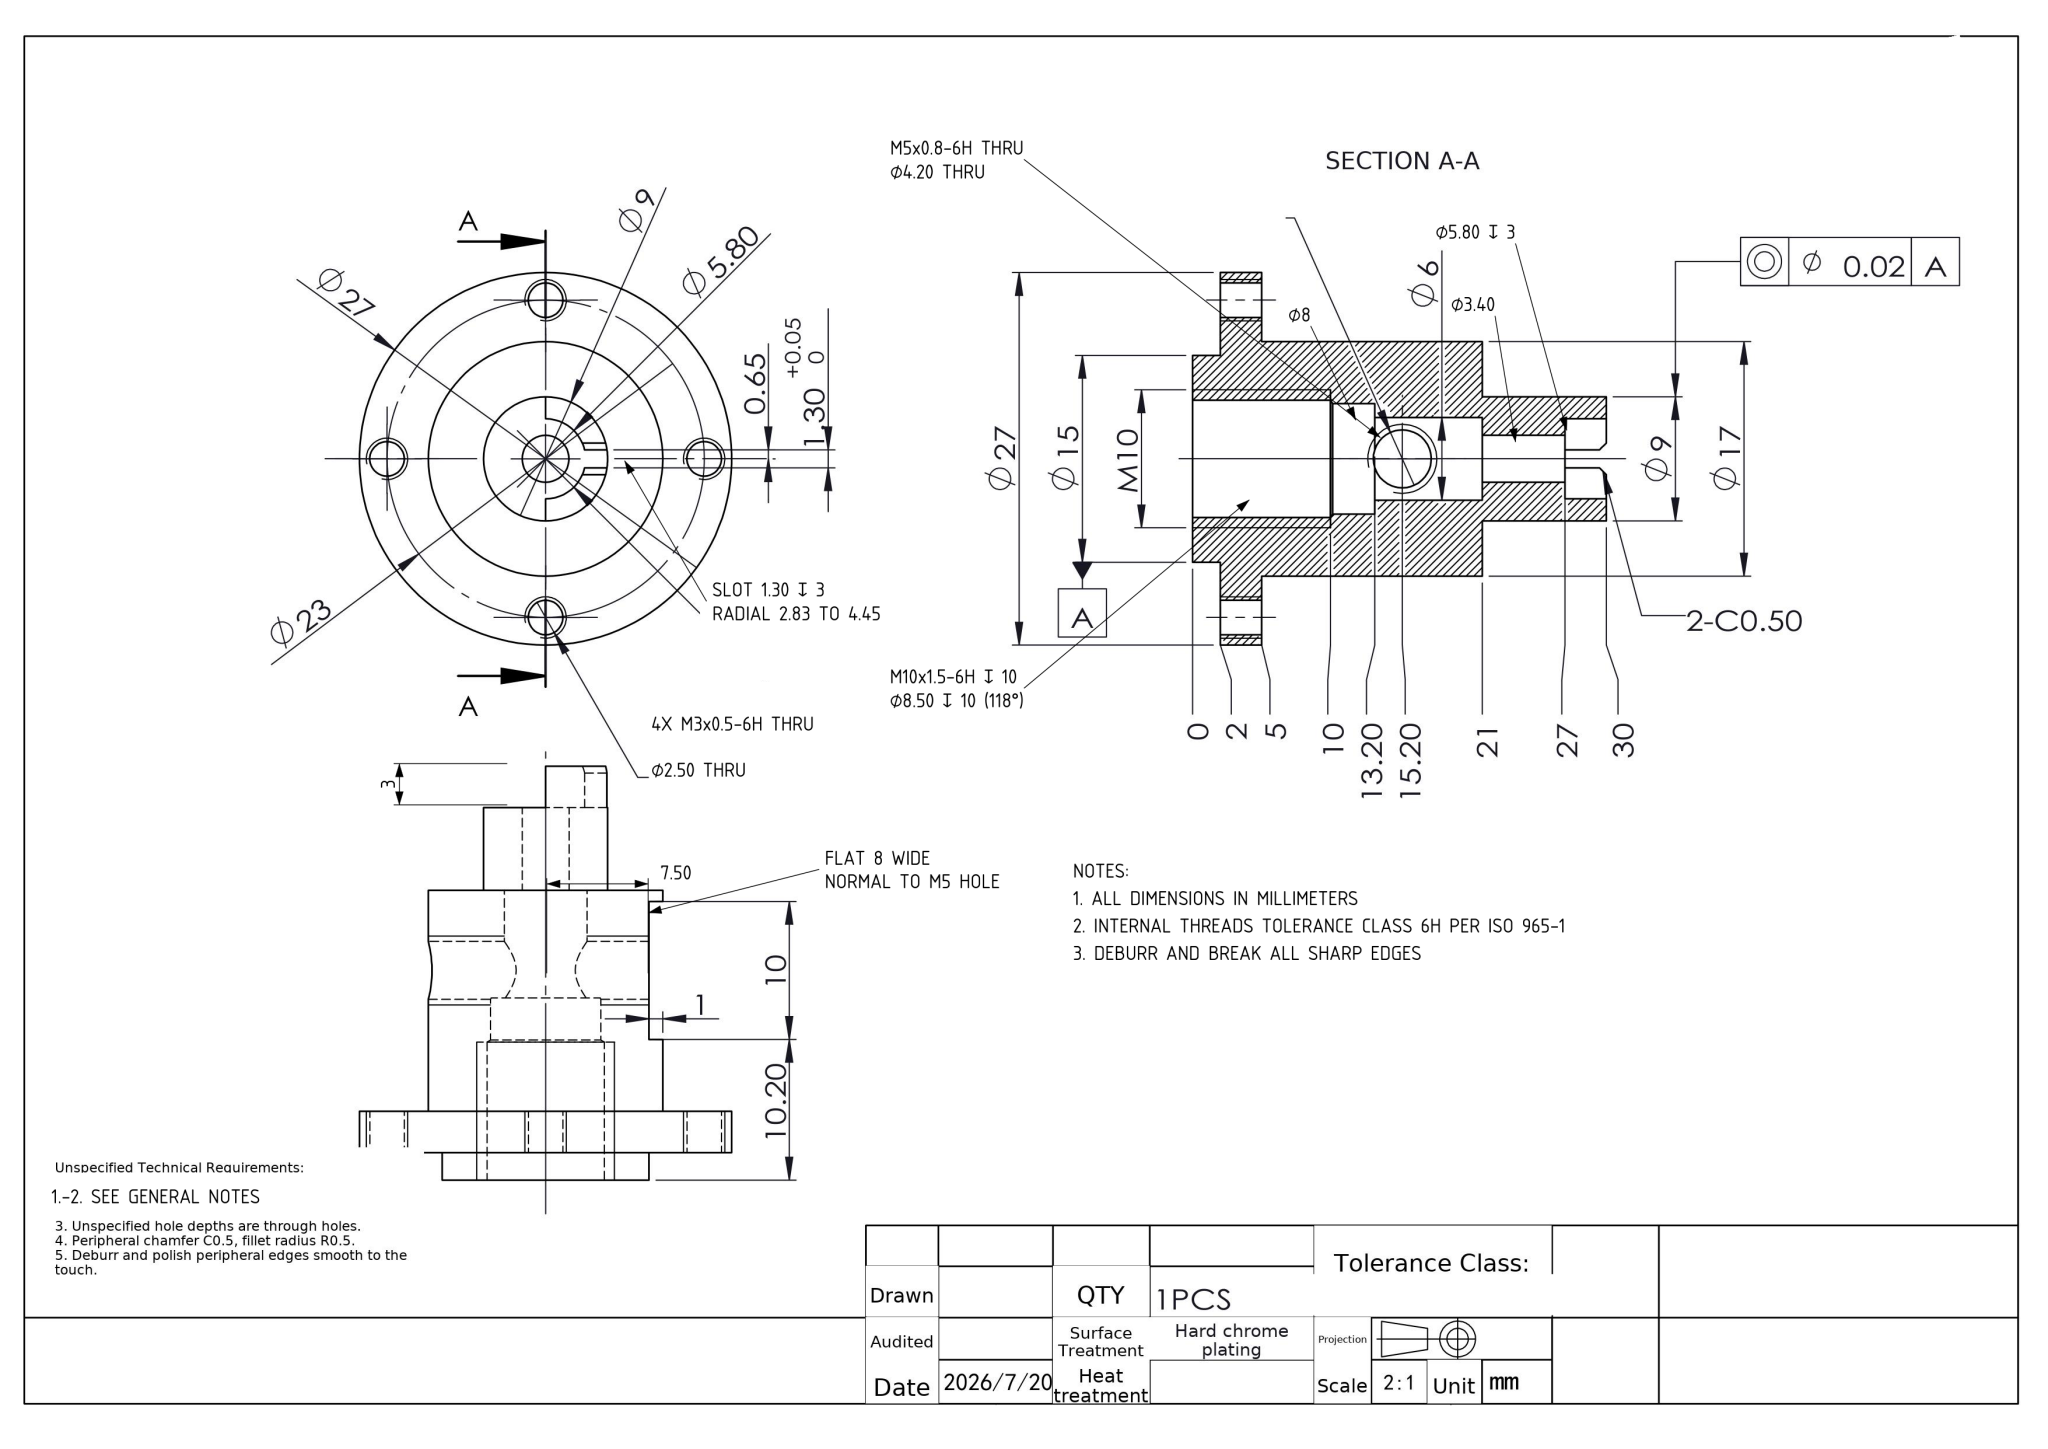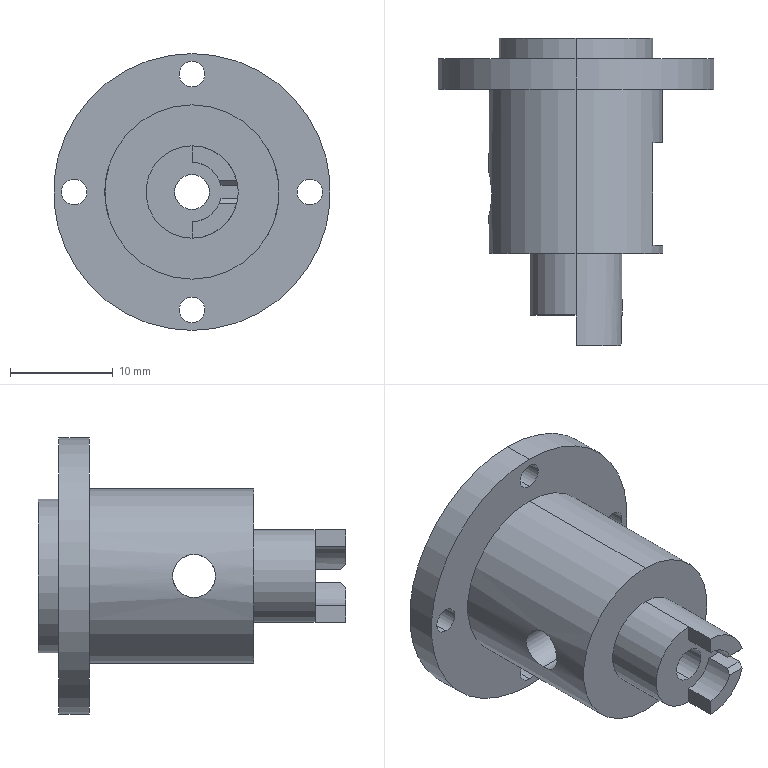Part | NX | mm | 1 solid | 51 faces | box 27 x 30 x 27 mm | volume 4874 mm3 | cylinder 30 | plane 19 | cone 2 | commonest cylinder face diameters 2.5 x8 4.2 x4 8.5 x2 6 x2 9 x2 8 x2 15 x2 27 x2